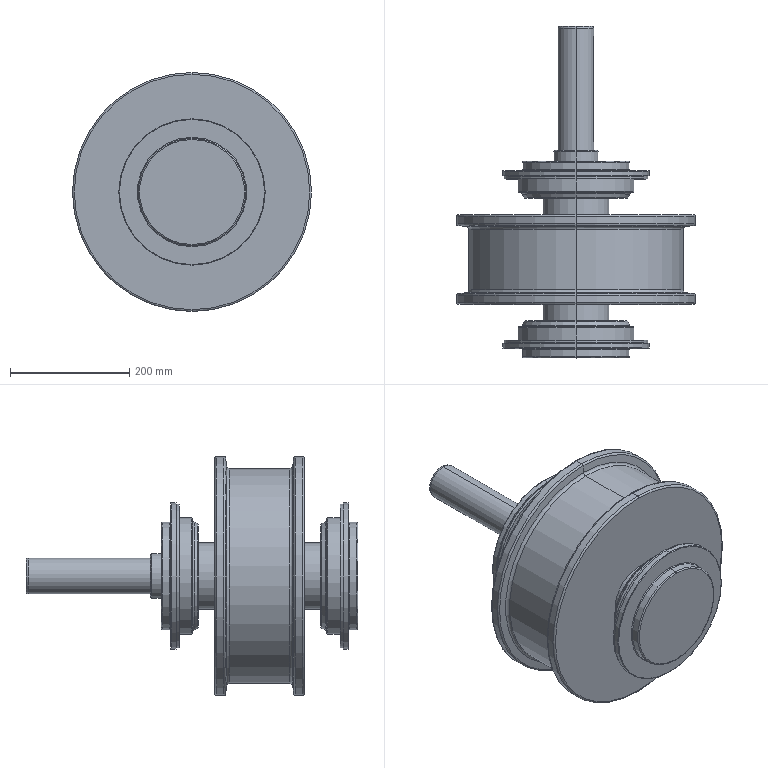Component | SolidWorks | WheelMain-3 | 1 solid | 104 faces | box 400 x 555.5 x 400 mm | volume 21306765 mm3 | torus 36 | cylinder 33 | plane 19 | cone 16 | commonest cylinder face diameters 180 x4 245 x4 240 x4 195 x4 112 x4 400 x4 18 x3 75 x2 | material Plain Carbon Steel
build123d program:
from build123d import *

# Parameters (mm, degrees)
CUT_EXTRUDE1_DEPTH      = 3
CUT_EXTRUDE1_DEPTH_BACK = 3
CUT_EXTRUDE1_START      = 29


with BuildPart() as part:
    # Sketch2 → Revolve1 (revolve)
    with BuildSketch(Plane.XY):
        with BuildLine():
            Line((0, 0), (0, 29))
            Line((0, 29), (-3.5, 30))
            Line((-3.5, 30), (-208, 30))
            Line((-208, 30), (-208, 35.5))
            Line((-208, 35.5), (-210, 37.5))
            Line((-210, 37.5), (-226.5, 37.5))
            Line((-226.5, 37.5), (-226.5, 88))
            ThreePointArc((-226.5, 88), (-227.086, 89.414), (-228.5, 90))
            Line((-228.5, 90), (-240.5, 90))
            ThreePointArc((-240.5, 90), (-241.561, 90.439), (-242, 91.5))
            Line((-242, 91.5), (-242, 121.5))
            ThreePointArc((-242, 121.5), (-242.293, 122.207), (-243, 122.5))
            Line((-243, 122.5), (-251, 122.5))
            Line((-251, 122.5), (-251, 120.5))
            ThreePointArc((-251, 120.5), (-251.146, 120.146), (-251.5, 120))
            Line((-251.5, 120), (-256, 120))
            Line((-256, 120), (-256, 97.5))
            Line((-256, 97.5), (-277, 97.5))
            Line((-277, 97.5), (-278.5, 96.5))
            Line((-278.5, 96.5), (-278.5, 94.474))
            ThreePointArc((-278.5, 94.474), (-279.237, 91.977), (-281.212, 90.279))
            Line((-281.212, 90.279), (-287.049, 87.653))
            ThreePointArc((-287.049, 87.653), (-288.106, 86.745), (-288.5, 85.409))
            Line((-288.5, 85.409), (-288.5, 56))
            Line((-288.5, 56), (-316, 56))
            Line((-316, 56), (-316, 197))
            ThreePointArc((-316, 197), (-316.879, 199.121), (-319, 200))
            Line((-319, 200), (-331.199, 200))
            ThreePointArc((-331.199, 200), (-333.206, 199.229), (-334.182, 197.313))
            Line((-334.182, 197.313), (-335.53, 184.478))
            ThreePointArc((-335.53, 184.478), (-337.157, 181.284), (-340.502, 180))
            Line((-340.502, 180), (-441.498, 180))
            ThreePointArc((-441.498, 180), (-444.843, 181.284), (-446.47, 184.478))
            Line((-446.47, 184.478), (-447.818, 197.313))
            ThreePointArc((-447.818, 197.313), (-448.794, 199.229), (-450.801, 200))
            Line((-450.801, 200), (-463, 200))
            ThreePointArc((-463, 200), (-465.121, 199.121), (-466, 197))
            Line((-466, 197), (-466, 56))
            Line((-466, 56), (-493.5, 56))
            Line((-493.5, 56), (-493.5, 85.409))
            ThreePointArc((-493.5, 85.409), (-493.894, 86.745), (-494.951, 87.653))
            Line((-494.951, 87.653), (-500.788, 90.279))
            ThreePointArc((-500.788, 90.279), (-502.763, 91.977), (-503.5, 94.474))
            Line((-503.5, 94.474), (-503.5, 96.5))
            Line((-503.5, 96.5), (-505, 97.5))
            Line((-505, 97.5), (-526, 97.5))
            Line((-526, 97.5), (-526, 120))
            Line((-526, 120), (-530.5, 120))
            ThreePointArc((-530.5, 120), (-530.854, 120.146), (-531, 120.5))
            Line((-531, 120.5), (-531, 122.5))
            Line((-531, 122.5), (-539, 122.5))
            ThreePointArc((-539, 122.5), (-539.707, 122.207), (-540, 121.5))
            Line((-540, 121.5), (-540, 91.5))
            ThreePointArc((-540, 91.5), (-540.439, 90.439), (-541.5, 90))
            Line((-541.5, 90), (-553.5, 90))
            ThreePointArc((-553.5, 90), (-554.914, 89.414), (-555.5, 88))
            Line((-555.5, 88), (-555.5, 0))
            Line((-555.5, 0), (0, 0))
        make_face()
    revolve(axis=Axis((0, 0, 0), (-1, 0, 0)))

    # Sketch3 → Cut-Extrude1 (cut, two sides: drawn at the far end of the back side and taken through both)
    with BuildSketch(Plane.XY.offset(CUT_EXTRUDE1_START - CUT_EXTRUDE1_DEPTH_BACK)):
        with BuildLine():
            Line((-186, 9), (-24, 9))
            ThreePointArc((-24, 9), (-15, 0), (-24, -9))
            Line((-24, -9), (-186, -9))
            ThreePointArc((-186, -9), (-195, 0), (-186, 9))
        make_face()
    extrude(amount=CUT_EXTRUDE1_DEPTH + CUT_EXTRUDE1_DEPTH_BACK, mode=Mode.SUBTRACT)


solid = part.part

# Placed as in the assembly
solid = solid.moved(Location((550.579, 1647.349, 2003.088), (90, 90, 0)))